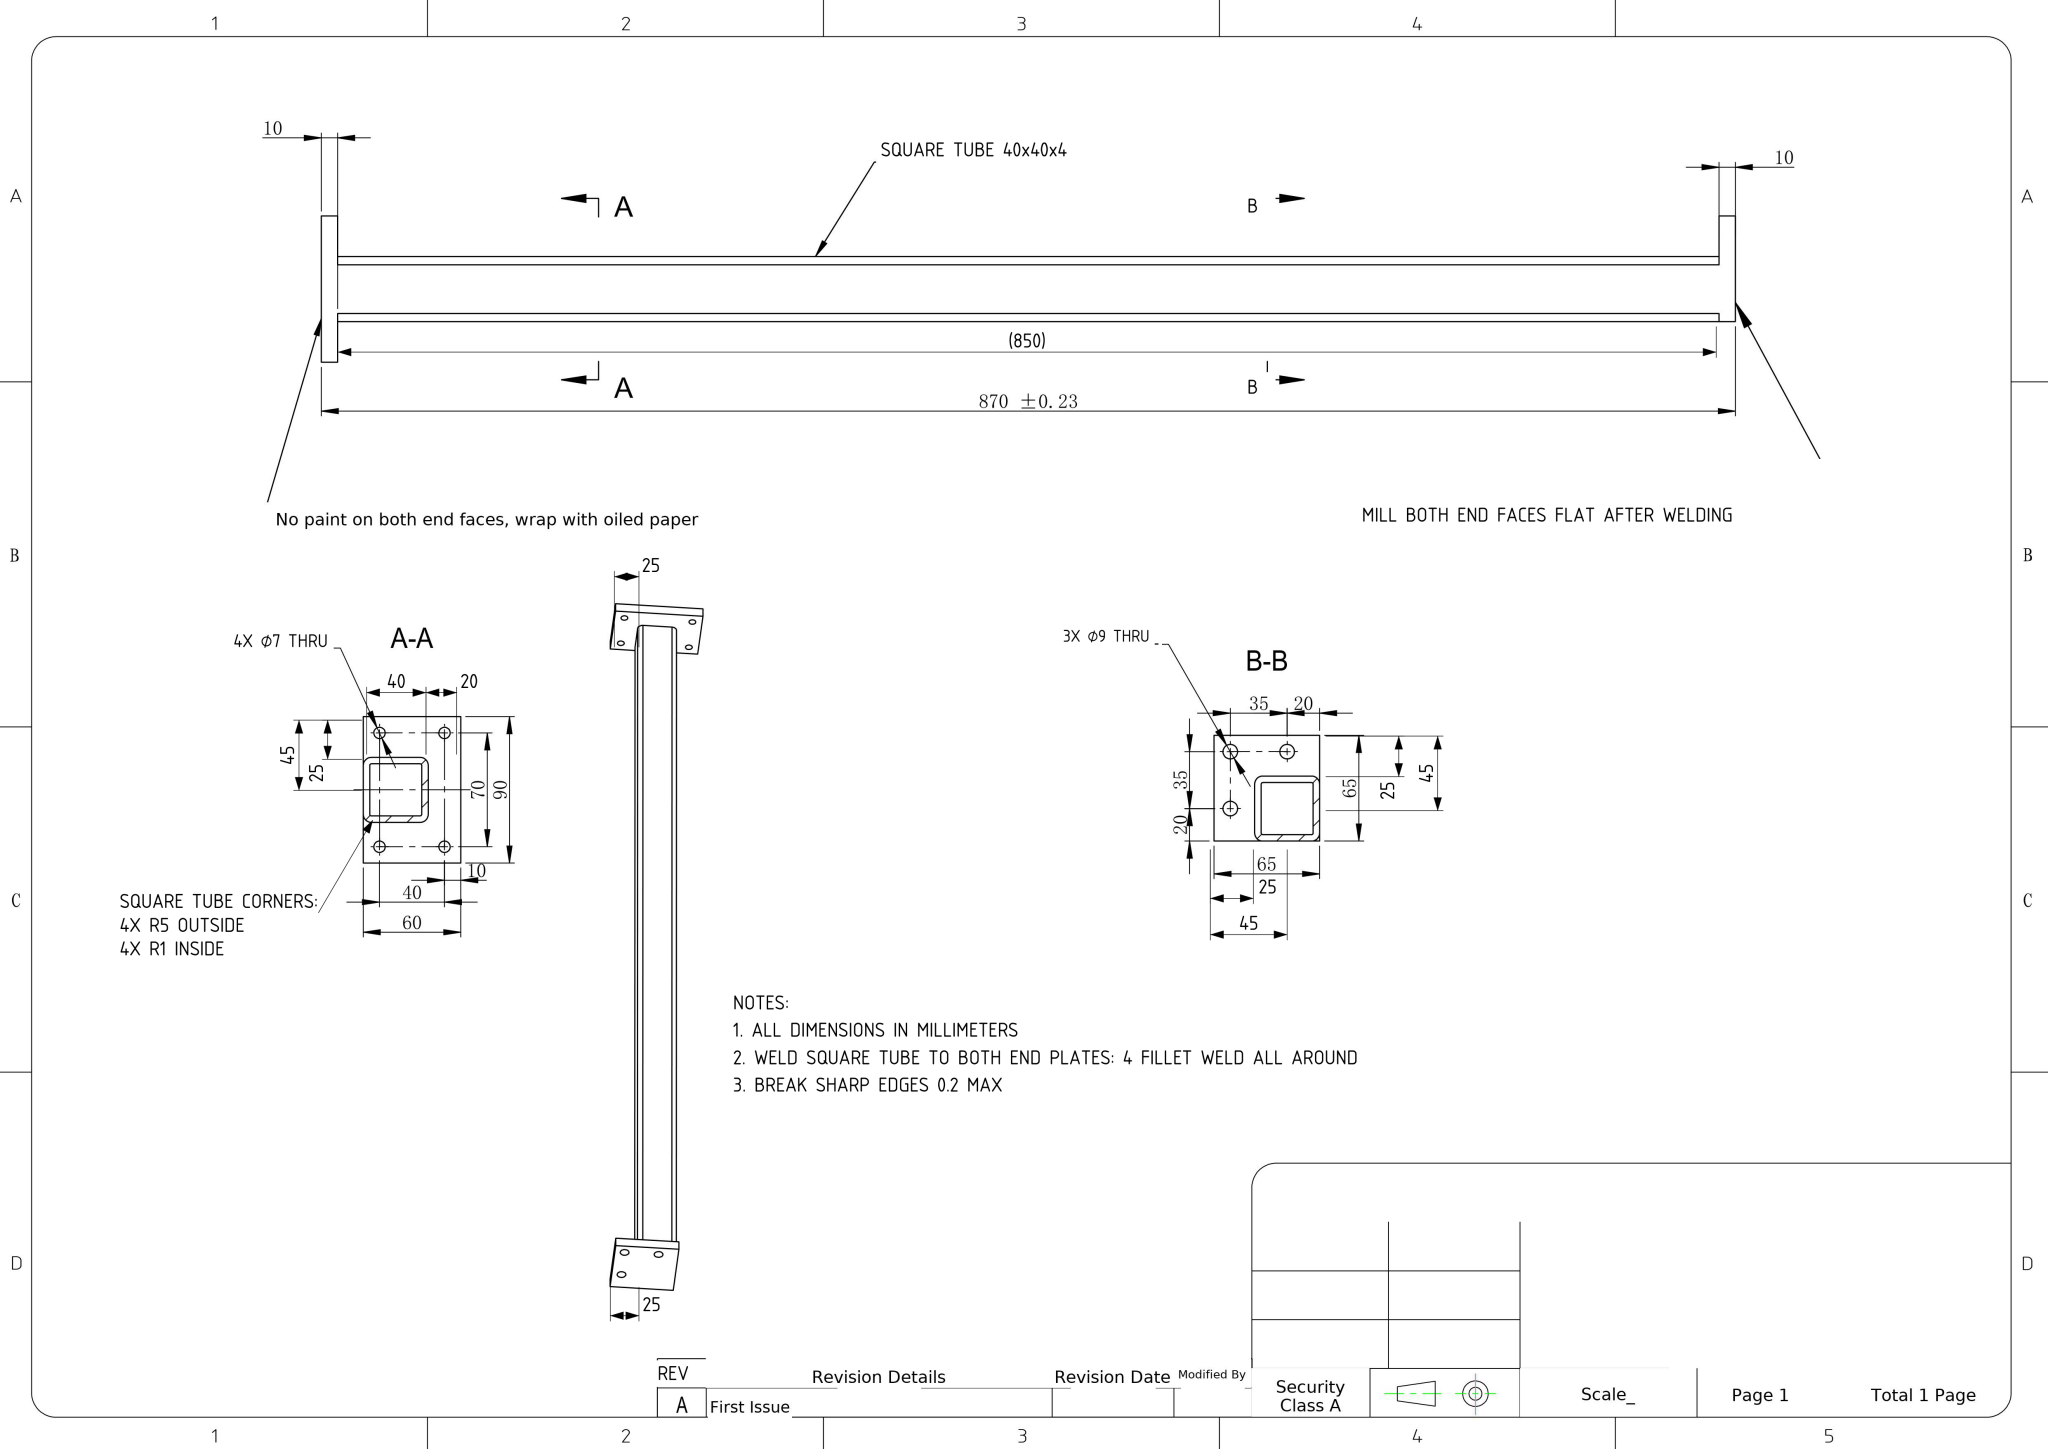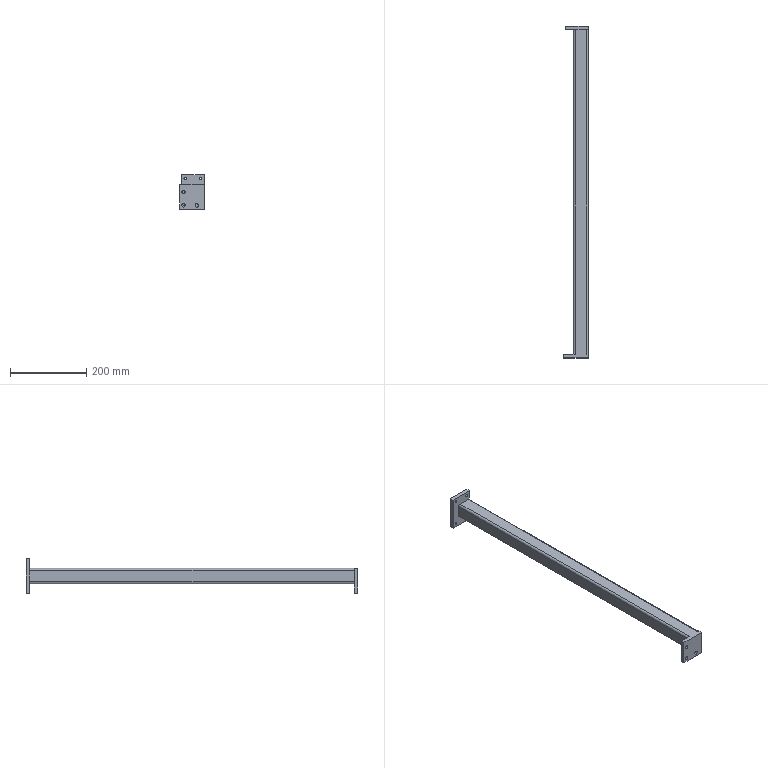Part | NX | mm | 1 solid | 42 faces | box 65 x 870 x 90 mm | volume 564891 mm3 | cylinder 22 | plane 20 | commonest cylinder face diameters 7 x8 9 x6 10 x4 2 x4